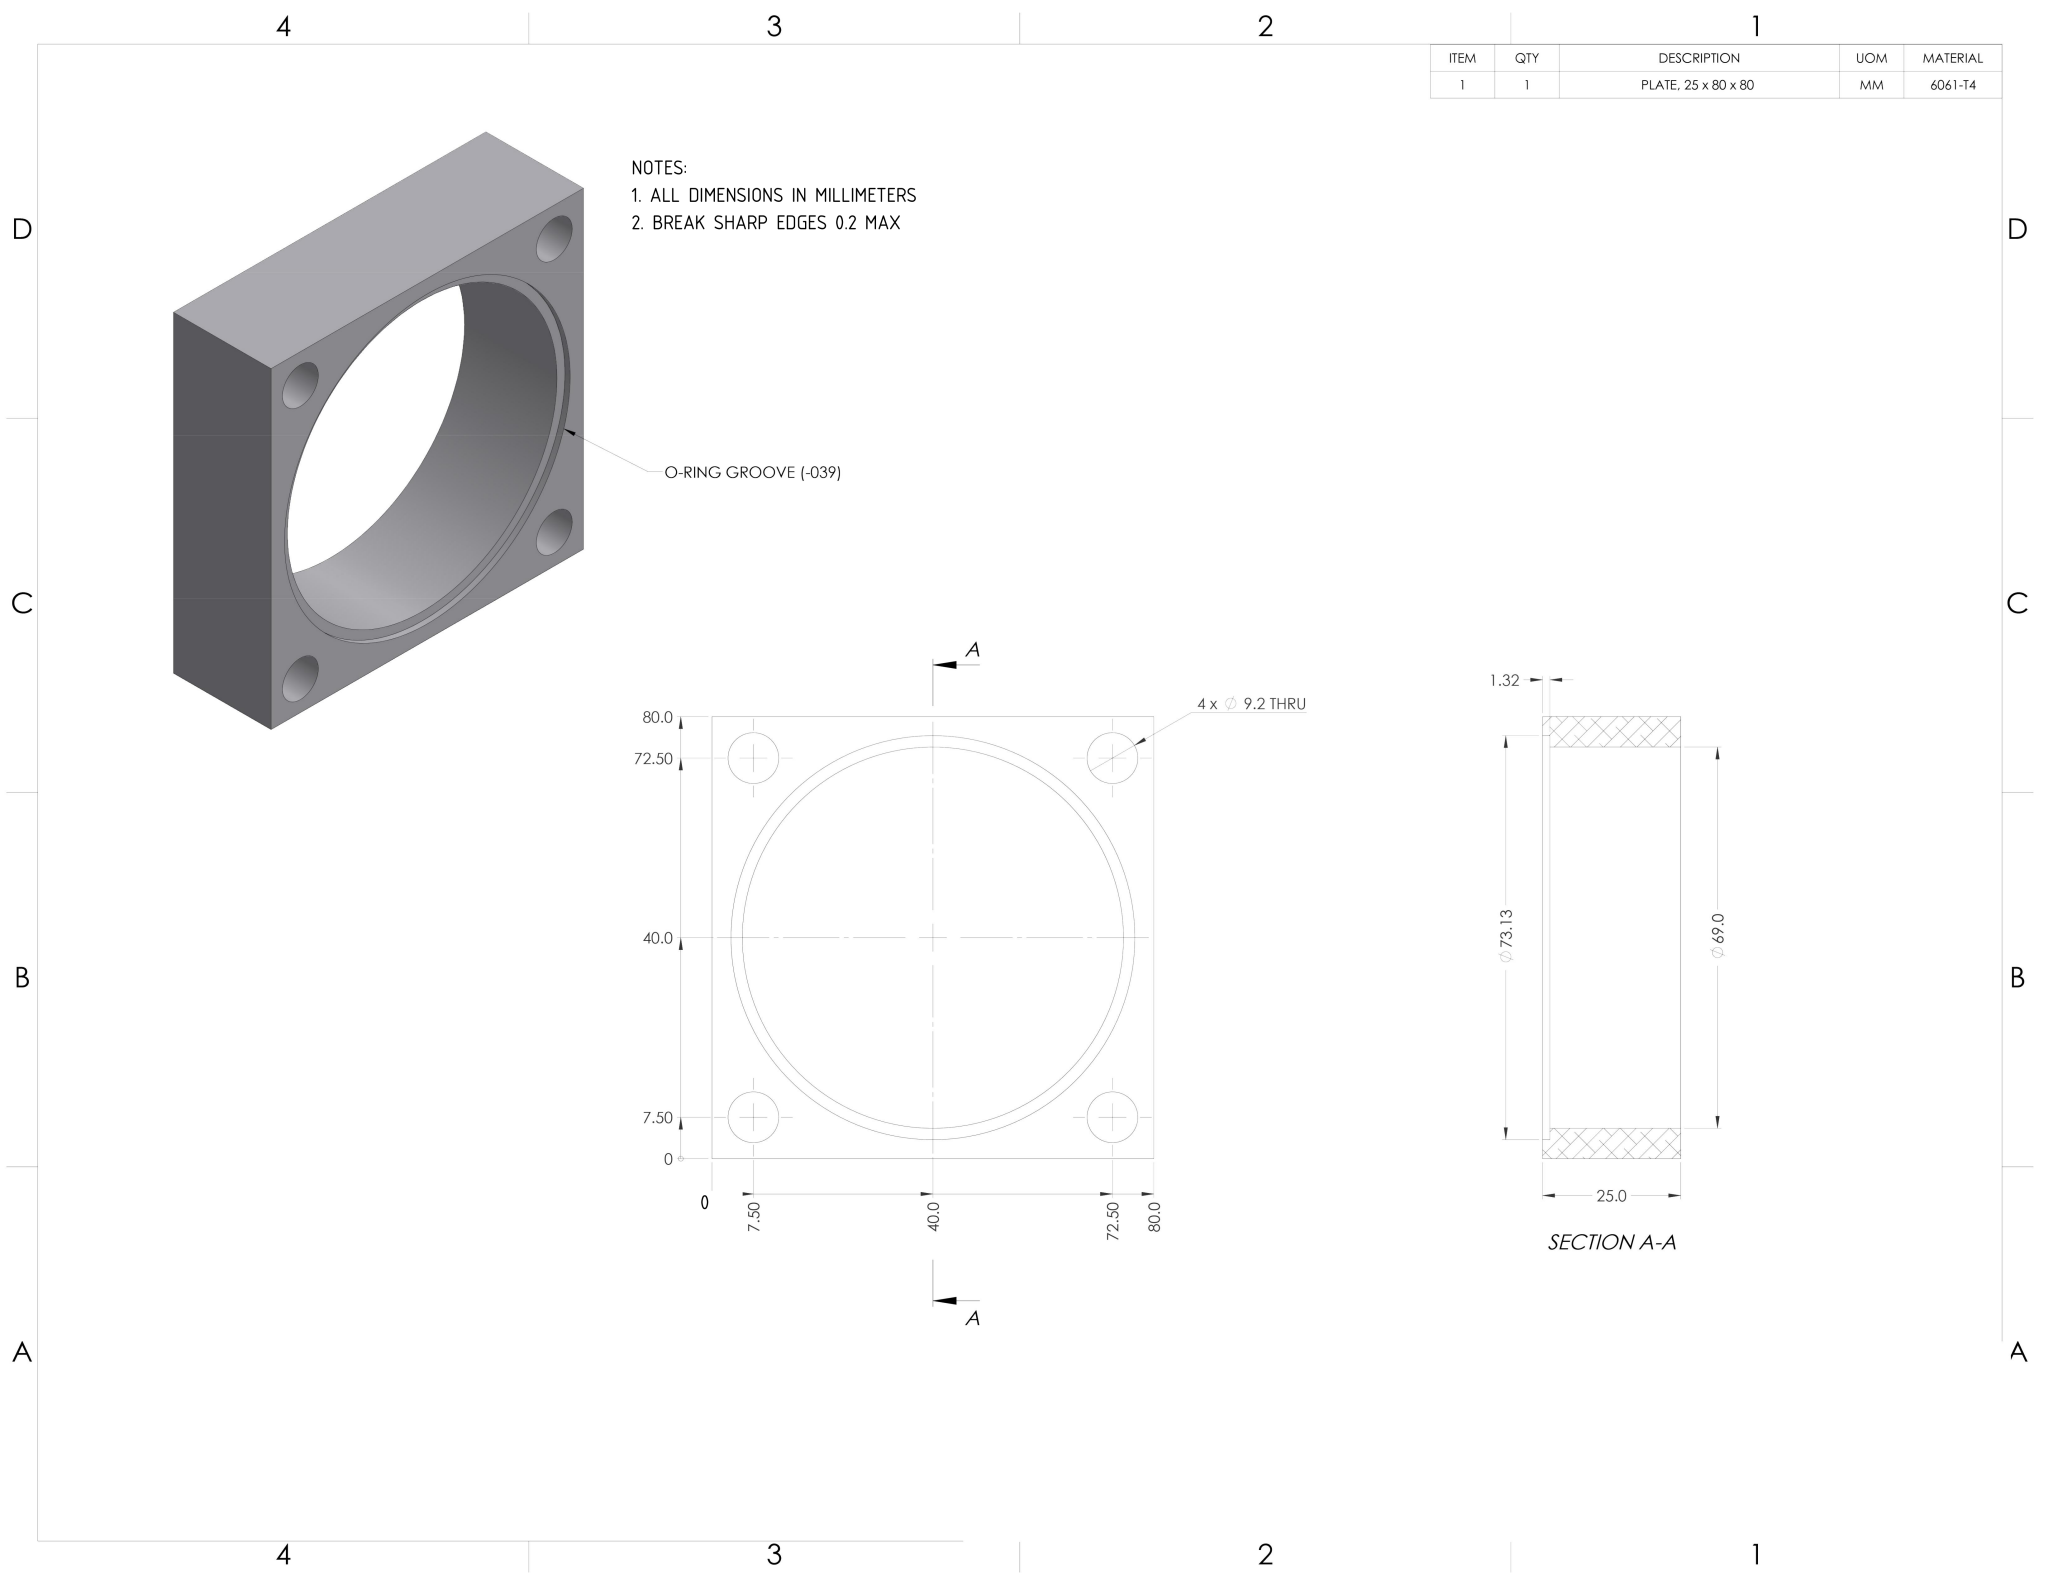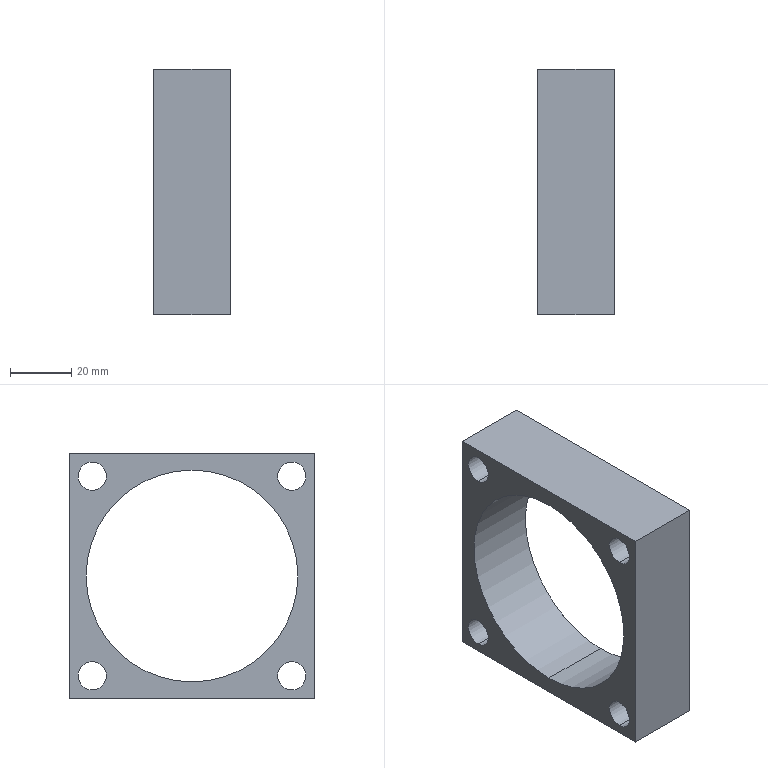Part | NX | mm | Four-Hole Circular Aperture Mounting Bracket | 1 solid | 19 faces | box 25 x 80 x 80 mm | volume 59262 mm3 | cylinder 12 | plane 7 | commonest cylinder face diameters 9.2 x8 69 x2 73.13 x2
STEP:
#1=COLOUR_RGB('',0.8667,0.8667,0.8902);
#2=FILL_AREA_STYLE_COLOUR('',#1);
#3=FILL_AREA_STYLE('',(#2));
#4=SURFACE_STYLE_FILL_AREA(#3);
#5=SURFACE_SIDE_STYLE('',(#4));
#6=SURFACE_STYLE_USAGE(.BOTH.,#5);
#7=PRESENTATION_STYLE_ASSIGNMENT((#6));
#8=CARTESIAN_POINT('',(11.18,0.,34.5));
#9=VERTEX_POINT('',#8);
#10=CARTESIAN_POINT('',(11.18,0.,-34.5));
#11=VERTEX_POINT('',#10);
#12=CARTESIAN_POINT('',(11.18,0.,0.));
#13=DIRECTION('',(1.,0.,0.));
#14=DIRECTION('',(0.,0.,-1.));
#15=AXIS2_PLACEMENT_3D('',#12,#13,#14);
#16=CIRCLE('',#15,34.5);
#17=EDGE_CURVE('',#9,#11,#16,.T.);
#18=ORIENTED_EDGE('',*,*,#17,.T.);
#19=CARTESIAN_POINT('',(-12.5,0.,-34.5));
#20=VERTEX_POINT('',#19);
#21=CARTESIAN_POINT('',(12.501,0.,-34.5));
#22=DIRECTION('',(-1.,0.,0.));
#23=VECTOR('',#22,1000.);
#24=LINE('',#21,#23);
#25=EDGE_CURVE('',#11,#20,#24,.T.);
#26=ORIENTED_EDGE('',*,*,#25,.T.);
#27=CARTESIAN_POINT('',(-12.5,0.,34.5));
#28=VERTEX_POINT('',#27);
#29=CARTESIAN_POINT('',(-12.5,0.,0.));
#30=DIRECTION('',(1.,0.,0.));
#31=DIRECTION('',(0.,0.,-1.));
#32=AXIS2_PLACEMENT_3D('',#29,#30,#31);
#33=CIRCLE('',#32,34.5);
#34=EDGE_CURVE('',#28,#20,#33,.T.);
#35=ORIENTED_EDGE('',*,*,#34,.F.);
#36=CARTESIAN_POINT('',(12.501,0.,34.5));
#37=DIRECTION('',(-1.,0.,0.));
#38=VECTOR('',#37,1000.);
#39=LINE('',#36,#38);
#40=EDGE_CURVE('',#9,#28,#39,.T.);
#41=ORIENTED_EDGE('',*,*,#40,.F.);
#42=EDGE_LOOP('',(#18,#26,#35,#41));
#43=FACE_OUTER_BOUND('',#42,.T.);
#44=CARTESIAN_POINT('',(12.501,0.,0.));
#45=DIRECTION('',(-1.,0.,0.));
#46=DIRECTION('',(0.,0.,1.));
#47=AXIS2_PLACEMENT_3D('',#44,#45,#46);
#48=CYLINDRICAL_SURFACE('',#47,34.5);
#49=ADVANCED_FACE('',(#43),#48,.F.);
#50=CARTESIAN_POINT('',(11.18,0.,36.565));
#51=VERTEX_POINT('',#50);
#52=CARTESIAN_POINT('',(11.18,0.,-36.565));
#53=VERTEX_POINT('',#52);
#54=CARTESIAN_POINT('',(11.18,0.,0.));
#55=DIRECTION('',(1.,0.,0.));
#56=DIRECTION('',(0.,0.,-1.));
#57=AXIS2_PLACEMENT_3D('',#54,#55,#56);
#58=CIRCLE('',#57,36.565);
#59=EDGE_CURVE('',#51,#53,#58,.T.);
#60=ORIENTED_EDGE('',*,*,#59,.F.);
#61=CARTESIAN_POINT('',(12.5,0.,36.565));
#62=VERTEX_POINT('',#61);
#63=CARTESIAN_POINT('',(11.18,0.,36.565));
#64=DIRECTION('',(1.,0.,0.));
#65=VECTOR('',#64,1000.);
#66=LINE('',#63,#65);
#67=EDGE_CURVE('',#51,#62,#66,.T.);
#68=ORIENTED_EDGE('',*,*,#67,.T.);
#69=CARTESIAN_POINT('',(12.5,0.,-36.565));
#70=VERTEX_POINT('',#69);
#71=CARTESIAN_POINT('',(12.5,0.,0.));
#72=DIRECTION('',(1.,0.,0.));
#73=DIRECTION('',(0.,0.,-1.));
#74=AXIS2_PLACEMENT_3D('',#71,#72,#73);
#75=CIRCLE('',#74,36.565);
#76=EDGE_CURVE('',#62,#70,#75,.T.);
#77=ORIENTED_EDGE('',*,*,#76,.T.);
#78=CARTESIAN_POINT('',(11.18,0.,-36.565));
#79=DIRECTION('',(1.,0.,0.));
#80=VECTOR('',#79,1000.);
#81=LINE('',#78,#80);
#82=EDGE_CURVE('',#53,#70,#81,.T.);
#83=ORIENTED_EDGE('',*,*,#82,.F.);
#84=EDGE_LOOP('',(#60,#68,#77,#83));
#85=FACE_OUTER_BOUND('',#84,.T.);
#86=CARTESIAN_POINT('',(11.18,0.,0.));
#87=DIRECTION('',(1.,0.,0.));
#88=DIRECTION('',(0.,0.,-1.));
#89=AXIS2_PLACEMENT_3D('',#86,#87,#88);
#90=CYLINDRICAL_SURFACE('',#89,36.565);
#91=ADVANCED_FACE('',(#85),#90,.F.);
#92=CARTESIAN_POINT('',(12.5,-32.5,37.1));
#93=VERTEX_POINT('',#92);
#94=CARTESIAN_POINT('',(12.5,-32.5,27.9));
#95=VERTEX_POINT('',#94);
#96=CARTESIAN_POINT('',(12.5,-32.5,32.5));
#97=DIRECTION('',(1.,0.,0.));
#98=DIRECTION('',(0.,0.,-1.));
#99=AXIS2_PLACEMENT_3D('',#96,#97,#98);
#100=CIRCLE('',#99,4.6);
#101=EDGE_CURVE('',#93,#95,#100,.T.);
#102=ORIENTED_EDGE('',*,*,#101,.T.);
#103=CARTESIAN_POINT('',(-12.5,-32.5,27.9));
#104=VERTEX_POINT('',#103);
#105=CARTESIAN_POINT('',(-12.5,-32.5,27.9));
#106=DIRECTION('',(-1.,0.,0.));
#107=VECTOR('',#106,1000.);
#108=LINE('',#105,#107);
#109=EDGE_CURVE('',#95,#104,#108,.T.);
#110=ORIENTED_EDGE('',*,*,#109,.T.);
#111=CARTESIAN_POINT('',(-12.5,-32.5,37.1));
#112=VERTEX_POINT('',#111);
#113=CARTESIAN_POINT('',(-12.5,-32.5,32.5));
#114=DIRECTION('',(-1.,0.,0.));
#115=DIRECTION('',(0.,0.,1.));
#116=AXIS2_PLACEMENT_3D('',#113,#114,#115);
#117=CIRCLE('',#116,4.6);
#118=EDGE_CURVE('',#104,#112,#117,.T.);
#119=ORIENTED_EDGE('',*,*,#118,.T.);
#120=CARTESIAN_POINT('',(-12.5,-32.5,37.1));
#121=DIRECTION('',(-1.,0.,0.));
#122=VECTOR('',#121,1000.);
#123=LINE('',#120,#122);
#124=EDGE_CURVE('',#93,#112,#123,.T.);
#125=ORIENTED_EDGE('',*,*,#124,.F.);
#126=EDGE_LOOP('',(#102,#110,#119,#125));
#127=FACE_OUTER_BOUND('',#126,.T.);
#128=CARTESIAN_POINT('',(-12.5,-32.5,32.5));
#129=DIRECTION('',(-1.,0.,0.));
#130=DIRECTION('',(0.,0.,1.));
#131=AXIS2_PLACEMENT_3D('',#128,#129,#130);
#132=CYLINDRICAL_SURFACE('',#131,4.6);
#133=ADVANCED_FACE('',(#127),#132,.F.);
#134=CARTESIAN_POINT('',(12.5,-32.5,-27.9));
#135=VERTEX_POINT('',#134);
#136=CARTESIAN_POINT('',(12.5,-32.5,-37.1));
#137=VERTEX_POINT('',#136);
#138=CARTESIAN_POINT('',(12.5,-32.5,-32.5));
#139=DIRECTION('',(1.,0.,0.));
#140=DIRECTION('',(0.,0.,-1.));
#141=AXIS2_PLACEMENT_3D('',#138,#139,#140);
#142=CIRCLE('',#141,4.6);
#143=EDGE_CURVE('',#135,#137,#142,.T.);
#144=ORIENTED_EDGE('',*,*,#143,.T.);
#145=CARTESIAN_POINT('',(-12.5,-32.5,-37.1));
#146=VERTEX_POINT('',#145);
#147=CARTESIAN_POINT('',(-12.5,-32.5,-37.1));
#148=DIRECTION('',(-1.,0.,0.));
#149=VECTOR('',#148,1000.);
#150=LINE('',#147,#149);
#151=EDGE_CURVE('',#137,#146,#150,.T.);
#152=ORIENTED_EDGE('',*,*,#151,.T.);
#153=CARTESIAN_POINT('',(-12.5,-32.5,-27.9));
#154=VERTEX_POINT('',#153);
#155=CARTESIAN_POINT('',(-12.5,-32.5,-32.5));
#156=DIRECTION('',(-1.,0.,0.));
#157=DIRECTION('',(0.,0.,1.));
#158=AXIS2_PLACEMENT_3D('',#155,#156,#157);
#159=CIRCLE('',#158,4.6);
#160=EDGE_CURVE('',#146,#154,#159,.T.);
#161=ORIENTED_EDGE('',*,*,#160,.T.);
#162=CARTESIAN_POINT('',(-12.5,-32.5,-27.9));
#163=DIRECTION('',(-1.,0.,0.));
#164=VECTOR('',#163,1000.);
#165=LINE('',#162,#164);
#166=EDGE_CURVE('',#135,#154,#165,.T.);
#167=ORIENTED_EDGE('',*,*,#166,.F.);
#168=EDGE_LOOP('',(#144,#152,#161,#167));
#169=FACE_OUTER_BOUND('',#168,.T.);
#170=CARTESIAN_POINT('',(-12.5,-32.5,-32.5));
#171=DIRECTION('',(-1.,0.,0.));
#172=DIRECTION('',(0.,0.,1.));
#173=AXIS2_PLACEMENT_3D('',#170,#171,#172);
#174=CYLINDRICAL_SURFACE('',#173,4.6);
#175=ADVANCED_FACE('',(#169),#174,.F.);
#176=CARTESIAN_POINT('',(12.5,32.5,-27.9));
#177=VERTEX_POINT('',#176);
#178=CARTESIAN_POINT('',(12.5,32.5,-37.1));
#179=VERTEX_POINT('',#178);
#180=CARTESIAN_POINT('',(12.5,32.5,-32.5));
#181=DIRECTION('',(1.,0.,0.));
#182=DIRECTION('',(0.,0.,-1.));
#183=AXIS2_PLACEMENT_3D('',#180,#181,#182);
#184=CIRCLE('',#183,4.6);
#185=EDGE_CURVE('',#177,#179,#184,.T.);
#186=ORIENTED_EDGE('',*,*,#185,.T.);
#187=CARTESIAN_POINT('',(-12.5,32.5,-37.1));
#188=VERTEX_POINT('',#187);
#189=CARTESIAN_POINT('',(-12.5,32.5,-37.1));
#190=DIRECTION('',(-1.,0.,0.));
#191=VECTOR('',#190,1000.);
#192=LINE('',#189,#191);
#193=EDGE_CURVE('',#179,#188,#192,.T.);
#194=ORIENTED_EDGE('',*,*,#193,.T.);
#195=CARTESIAN_POINT('',(-12.5,32.5,-27.9));
#196=VERTEX_POINT('',#195);
#197=CARTESIAN_POINT('',(-12.5,32.5,-32.5));
#198=DIRECTION('',(-1.,0.,0.));
#199=DIRECTION('',(0.,0.,1.));
#200=AXIS2_PLACEMENT_3D('',#197,#198,#199);
#201=CIRCLE('',#200,4.6);
#202=EDGE_CURVE('',#188,#196,#201,.T.);
#203=ORIENTED_EDGE('',*,*,#202,.T.);
#204=CARTESIAN_POINT('',(-12.5,32.5,-27.9));
#205=DIRECTION('',(-1.,0.,0.));
#206=VECTOR('',#205,1000.);
#207=LINE('',#204,#206);
#208=EDGE_CURVE('',#177,#196,#207,.T.);
#209=ORIENTED_EDGE('',*,*,#208,.F.);
#210=EDGE_LOOP('',(#186,#194,#203,#209));
#211=FACE_OUTER_BOUND('',#210,.T.);
#212=CARTESIAN_POINT('',(-12.5,32.5,-32.5));
#213=DIRECTION('',(-1.,0.,0.));
#214=DIRECTION('',(0.,0.,1.));
#215=AXIS2_PLACEMENT_3D('',#212,#213,#214);
#216=CYLINDRICAL_SURFACE('',#215,4.6);
#217=ADVANCED_FACE('',(#211),#216,.F.);
#218=CARTESIAN_POINT('',(12.5,32.5,37.1));
#219=VERTEX_POINT('',#218);
#220=CARTESIAN_POINT('',(12.5,32.5,27.9));
#221=VERTEX_POINT('',#220);
#222=CARTESIAN_POINT('',(12.5,32.5,32.5));
#223=DIRECTION('',(1.,0.,0.));
#224=DIRECTION('',(0.,0.,-1.));
#225=AXIS2_PLACEMENT_3D('',#222,#223,#224);
#226=CIRCLE('',#225,4.6);
#227=EDGE_CURVE('',#219,#221,#226,.T.);
#228=ORIENTED_EDGE('',*,*,#227,.T.);
#229=CARTESIAN_POINT('',(-12.5,32.5,27.9));
#230=VERTEX_POINT('',#229);
#231=CARTESIAN_POINT('',(-12.5,32.5,27.9));
#232=DIRECTION('',(-1.,0.,0.));
#233=VECTOR('',#232,1000.);
#234=LINE('',#231,#233);
#235=EDGE_CURVE('',#221,#230,#234,.T.);
#236=ORIENTED_EDGE('',*,*,#235,.T.);
#237=CARTESIAN_POINT('',(-12.5,32.5,37.1));
#238=VERTEX_POINT('',#237);
#239=CARTESIAN_POINT('',(-12.5,32.5,32.5));
#240=DIRECTION('',(-1.,0.,0.));
#241=DIRECTION('',(0.,0.,1.));
#242=AXIS2_PLACEMENT_3D('',#239,#240,#241);
#243=CIRCLE('',#242,4.6);
#244=EDGE_CURVE('',#230,#238,#243,.T.);
#245=ORIENTED_EDGE('',*,*,#244,.T.);
#246=CARTESIAN_POINT('',(-12.5,32.5,37.1));
#247=DIRECTION('',(-1.,0.,0.));
#248=VECTOR('',#247,1000.);
#249=LINE('',#246,#248);
#250=EDGE_CURVE('',#219,#238,#249,.T.);
#251=ORIENTED_EDGE('',*,*,#250,.F.);
#252=EDGE_LOOP('',(#228,#236,#245,#251));
#253=FACE_OUTER_BOUND('',#252,.T.);
#254=CARTESIAN_POINT('',(-12.5,32.5,32.5));
#255=DIRECTION('',(-1.,0.,0.));
#256=DIRECTION('',(0.,0.,1.));
#257=AXIS2_PLACEMENT_3D('',#254,#255,#256);
#258=CYLINDRICAL_SURFACE('',#257,4.6);
#259=ADVANCED_FACE('',(#253),#258,.F.);
#260=ORIENTED_EDGE('',*,*,#34,.T.);
#261=CARTESIAN_POINT('',(-12.5,0.,0.));
#262=DIRECTION('',(1.,0.,0.));
#263=DIRECTION('',(0.,0.,-1.));
#264=AXIS2_PLACEMENT_3D('',#261,#262,#263);
#265=CIRCLE('',#264,34.5);
#266=EDGE_CURVE('',#20,#28,#265,.T.);
#267=ORIENTED_EDGE('',*,*,#266,.T.);
#268=EDGE_LOOP('',(#260,#267));
#269=FACE_BOUND('',#268,.T.);
#270=CARTESIAN_POINT('',(-12.5,-32.5,-32.5));
#271=DIRECTION('',(-1.,0.,0.));
#272=DIRECTION('',(0.,0.,1.));
#273=AXIS2_PLACEMENT_3D('',#270,#271,#272);
#274=CIRCLE('',#273,4.6);
#275=EDGE_CURVE('',#154,#146,#274,.T.);
#276=ORIENTED_EDGE('',*,*,#275,.F.);
#277=ORIENTED_EDGE('',*,*,#160,.F.);
#278=EDGE_LOOP('',(#276,#277));
#279=FACE_BOUND('',#278,.T.);
#280=CARTESIAN_POINT('',(-12.5,32.5,-32.5));
#281=DIRECTION('',(-1.,0.,0.));
#282=DIRECTION('',(0.,0.,1.));
#283=AXIS2_PLACEMENT_3D('',#280,#281,#282);
#284=CIRCLE('',#283,4.6);
#285=EDGE_CURVE('',#196,#188,#284,.T.);
#286=ORIENTED_EDGE('',*,*,#285,.F.);
#287=ORIENTED_EDGE('',*,*,#202,.F.);
#288=EDGE_LOOP('',(#286,#287));
#289=FACE_BOUND('',#288,.T.);
#290=CARTESIAN_POINT('',(-12.5,32.5,32.5));
#291=DIRECTION('',(-1.,0.,0.));
#292=DIRECTION('',(0.,0.,1.));
#293=AXIS2_PLACEMENT_3D('',#290,#291,#292);
#294=CIRCLE('',#293,4.6);
#295=EDGE_CURVE('',#238,#230,#294,.T.);
#296=ORIENTED_EDGE('',*,*,#295,.F.);
#297=ORIENTED_EDGE('',*,*,#244,.F.);
#298=EDGE_LOOP('',(#296,#297));
#299=FACE_BOUND('',#298,.T.);
#300=CARTESIAN_POINT('',(-12.5,40.,40.));
#301=VERTEX_POINT('',#300);
#302=CARTESIAN_POINT('',(-12.5,-40.,40.));
#303=VERTEX_POINT('',#302);
#304=CARTESIAN_POINT('',(-12.5,40.,40.));
#305=DIRECTION('',(0.,-1.,-0.));
#306=VECTOR('',#305,1000.);
#307=LINE('',#304,#306);
#308=EDGE_CURVE('',#301,#303,#307,.T.);
#309=ORIENTED_EDGE('',*,*,#308,.F.);
#310=CARTESIAN_POINT('',(-12.5,40.,-40.));
#311=VERTEX_POINT('',#310);
#312=CARTESIAN_POINT('',(-12.5,40.,40.));
#313=DIRECTION('',(0.,0.,1.));
#314=VECTOR('',#313,1000.);
#315=LINE('',#312,#314);
#316=EDGE_CURVE('',#311,#301,#315,.T.);
#317=ORIENTED_EDGE('',*,*,#316,.F.);
#318=CARTESIAN_POINT('',(-12.5,-40.,-40.));
#319=VERTEX_POINT('',#318);
#320=CARTESIAN_POINT('',(-12.5,40.,-40.));
#321=DIRECTION('',(0.,1.,-0.));
#322=VECTOR('',#321,1000.);
#323=LINE('',#320,#322);
#324=EDGE_CURVE('',#319,#311,#323,.T.);
#325=ORIENTED_EDGE('',*,*,#324,.F.);
#326=CARTESIAN_POINT('',(-12.5,-40.,40.));
#327=DIRECTION('',(0.,0.,-1.));
#328=VECTOR('',#327,1000.);
#329=LINE('',#326,#328);
#330=EDGE_CURVE('',#303,#319,#329,.T.);
#331=ORIENTED_EDGE('',*,*,#330,.F.);
#332=EDGE_LOOP('',(#309,#317,#325,#331));
#333=FACE_OUTER_BOUND('',#332,.T.);
#334=CARTESIAN_POINT('',(-12.5,-32.5,32.5));
#335=DIRECTION('',(-1.,0.,0.));
#336=DIRECTION('',(0.,0.,1.));
#337=AXIS2_PLACEMENT_3D('',#334,#335,#336);
#338=CIRCLE('',#337,4.6);
#339=EDGE_CURVE('',#112,#104,#338,.T.);
#340=ORIENTED_EDGE('',*,*,#339,.F.);
#341=ORIENTED_EDGE('',*,*,#118,.F.);
#342=EDGE_LOOP('',(#340,#341));
#343=FACE_BOUND('',#342,.T.);
#344=CARTESIAN_POINT('',(-12.5,0.,0.));
#345=DIRECTION('',(1.,0.,0.));
#346=DIRECTION('',(0.,0.,-1.));
#347=AXIS2_PLACEMENT_3D('',#344,#345,#346);
#348=PLANE('',#347);
#349=ADVANCED_FACE('',(#269,#279,#289,#299,#333,#343),#348,.F.);
#350=ORIENTED_EDGE('',*,*,#308,.T.);
#351=CARTESIAN_POINT('',(12.5,-40.,40.));
#352=VERTEX_POINT('',#351);
#353=CARTESIAN_POINT('',(12.5,-40.,40.));
#354=DIRECTION('',(-1.,0.,0.));
#355=VECTOR('',#354,1000.);
#356=LINE('',#353,#355);
#357=EDGE_CURVE('',#352,#303,#356,.T.);
#358=ORIENTED_EDGE('',*,*,#357,.F.);
#359=CARTESIAN_POINT('',(12.5,40.,40.));
#360=VERTEX_POINT('',#359);
#361=CARTESIAN_POINT('',(12.5,40.,40.));
#362=DIRECTION('',(0.,-1.,-0.));
#363=VECTOR('',#362,1000.);
#364=LINE('',#361,#363);
#365=EDGE_CURVE('',#360,#352,#364,.T.);
#366=ORIENTED_EDGE('',*,*,#365,.F.);
#367=CARTESIAN_POINT('',(12.5,40.,40.));
#368=DIRECTION('',(-1.,0.,0.));
#369=VECTOR('',#368,1000.);
#370=LINE('',#367,#369);
#371=EDGE_CURVE('',#360,#301,#370,.T.);
#372=ORIENTED_EDGE('',*,*,#371,.T.);
#373=EDGE_LOOP('',(#350,#358,#366,#372));
#374=FACE_OUTER_BOUND('',#373,.T.);
#375=CARTESIAN_POINT('',(12.5,40.,40.));
#376=DIRECTION('',(0.,0.,-1.));
#377=DIRECTION('',(0.,1.,0.));
#378=AXIS2_PLACEMENT_3D('',#375,#376,#377);
#379=PLANE('',#378);
#380=ADVANCED_FACE('',(#374),#379,.F.);
#381=ORIENTED_EDGE('',*,*,#330,.T.);
#382=CARTESIAN_POINT('',(12.5,-40.,-40.));
#383=VERTEX_POINT('',#382);
#384=CARTESIAN_POINT('',(12.5,-40.,-40.));
#385=DIRECTION('',(-1.,0.,0.));
#386=VECTOR('',#385,1000.);
#387=LINE('',#384,#386);
#388=EDGE_CURVE('',#383,#319,#387,.T.);
#389=ORIENTED_EDGE('',*,*,#388,.F.);
#390=CARTESIAN_POINT('',(12.5,-40.,40.));
#391=DIRECTION('',(0.,0.,-1.));
#392=VECTOR('',#391,1000.);
#393=LINE('',#390,#392);
#394=EDGE_CURVE('',#352,#383,#393,.T.);
#395=ORIENTED_EDGE('',*,*,#394,.F.);
#396=ORIENTED_EDGE('',*,*,#357,.T.);
#397=EDGE_LOOP('',(#381,#389,#395,#396));
#398=FACE_OUTER_BOUND('',#397,.T.);
#399=CARTESIAN_POINT('',(12.5,-40.,40.));
#400=DIRECTION('',(0.,1.,0.));
#401=DIRECTION('',(0.,0.,1.));
#402=AXIS2_PLACEMENT_3D('',#399,#400,#401);
#403=PLANE('',#402);
#404=ADVANCED_FACE('',(#398),#403,.F.);
#405=ORIENTED_EDGE('',*,*,#324,.T.);
#406=CARTESIAN_POINT('',(12.5,40.,-40.));
#407=VERTEX_POINT('',#406);
#408=CARTESIAN_POINT('',(12.5,40.,-40.));
#409=DIRECTION('',(-1.,0.,0.));
#410=VECTOR('',#409,1000.);
#411=LINE('',#408,#410);
#412=EDGE_CURVE('',#407,#311,#411,.T.);
#413=ORIENTED_EDGE('',*,*,#412,.F.);
#414=CARTESIAN_POINT('',(12.5,40.,-40.));
#415=DIRECTION('',(0.,1.,-0.));
#416=VECTOR('',#415,1000.);
#417=LINE('',#414,#416);
#418=EDGE_CURVE('',#383,#407,#417,.T.);
#419=ORIENTED_EDGE('',*,*,#418,.F.);
#420=ORIENTED_EDGE('',*,*,#388,.T.);
#421=EDGE_LOOP('',(#405,#413,#419,#420));
#422=FACE_OUTER_BOUND('',#421,.T.);
#423=CARTESIAN_POINT('',(12.5,40.,-40.));
#424=DIRECTION('',(0.,0.,1.));
#425=DIRECTION('',(0.,-1.,0.));
#426=AXIS2_PLACEMENT_3D('',#423,#424,#425);
#427=PLANE('',#426);
#428=ADVANCED_FACE('',(#422),#427,.F.);
#429=ORIENTED_EDGE('',*,*,#316,.T.);
#430=ORIENTED_EDGE('',*,*,#371,.F.);
#431=CARTESIAN_POINT('',(12.5,40.,40.));
#432=DIRECTION('',(0.,0.,1.));
#433=VECTOR('',#432,1000.);
#434=LINE('',#431,#433);
#435=EDGE_CURVE('',#407,#360,#434,.T.);
#436=ORIENTED_EDGE('',*,*,#435,.F.);
#437=ORIENTED_EDGE('',*,*,#412,.T.);
#438=EDGE_LOOP('',(#429,#430,#436,#437));
#439=FACE_OUTER_BOUND('',#438,.T.);
#440=CARTESIAN_POINT('',(12.5,40.,40.));
#441=DIRECTION('',(0.,-1.,0.));
#442=DIRECTION('',(0.,0.,-1.));
#443=AXIS2_PLACEMENT_3D('',#440,#441,#442);
#444=PLANE('',#443);
#445=ADVANCED_FACE('',(#439),#444,.F.);
#446=CARTESIAN_POINT('',(12.5,0.,0.));
#447=DIRECTION('',(1.,0.,0.));
#448=DIRECTION('',(0.,0.,-1.));
#449=AXIS2_PLACEMENT_3D('',#446,#447,#448);
#450=CIRCLE('',#449,36.565);
#451=EDGE_CURVE('',#70,#62,#450,.T.);
#452=ORIENTED_EDGE('',*,*,#451,.F.);
#453=ORIENTED_EDGE('',*,*,#76,.F.);
#454=EDGE_LOOP('',(#452,#453));
#455=FACE_BOUND('',#454,.T.);
#456=ORIENTED_EDGE('',*,*,#101,.F.);
#457=CARTESIAN_POINT('',(12.5,-32.5,32.5));
#458=DIRECTION('',(1.,0.,0.));
#459=DIRECTION('',(0.,0.,-1.));
#460=AXIS2_PLACEMENT_3D('',#457,#458,#459);
#461=CIRCLE('',#460,4.6);
#462=EDGE_CURVE('',#95,#93,#461,.T.);
#463=ORIENTED_EDGE('',*,*,#462,.F.);
#464=EDGE_LOOP('',(#456,#463));
#465=FACE_BOUND('',#464,.T.);
#466=ORIENTED_EDGE('',*,*,#143,.F.);
#467=CARTESIAN_POINT('',(12.5,-32.5,-32.5));
#468=DIRECTION('',(1.,0.,0.));
#469=DIRECTION('',(0.,0.,-1.));
#470=AXIS2_PLACEMENT_3D('',#467,#468,#469);
#471=CIRCLE('',#470,4.6);
#472=EDGE_CURVE('',#137,#135,#471,.T.);
#473=ORIENTED_EDGE('',*,*,#472,.F.);
#474=EDGE_LOOP('',(#466,#473));
#475=FACE_BOUND('',#474,.T.);
#476=ORIENTED_EDGE('',*,*,#185,.F.);
#477=CARTESIAN_POINT('',(12.5,32.5,-32.5));
#478=DIRECTION('',(1.,0.,0.));
#479=DIRECTION('',(0.,0.,-1.));
#480=AXIS2_PLACEMENT_3D('',#477,#478,#479);
#481=CIRCLE('',#480,4.6);
#482=EDGE_CURVE('',#179,#177,#481,.T.);
#483=ORIENTED_EDGE('',*,*,#482,.F.);
#484=EDGE_LOOP('',(#476,#483));
#485=FACE_BOUND('',#484,.T.);
#486=ORIENTED_EDGE('',*,*,#227,.F.);
#487=CARTESIAN_POINT('',(12.5,32.5,32.5));
#488=DIRECTION('',(1.,0.,0.));
#489=DIRECTION('',(0.,0.,-1.));
#490=AXIS2_PLACEMENT_3D('',#487,#488,#489);
#491=CIRCLE('',#490,4.6);
#492=EDGE_CURVE('',#221,#219,#491,.T.);
#493=ORIENTED_EDGE('',*,*,#492,.F.);
#494=EDGE_LOOP('',(#486,#493));
#495=FACE_BOUND('',#494,.T.);
#496=ORIENTED_EDGE('',*,*,#365,.T.);
#497=ORIENTED_EDGE('',*,*,#394,.T.);
#498=ORIENTED_EDGE('',*,*,#418,.T.);
#499=ORIENTED_EDGE('',*,*,#435,.T.);
#500=EDGE_LOOP('',(#496,#497,#498,#499));
#501=FACE_OUTER_BOUND('',#500,.T.);
#502=CARTESIAN_POINT('',(12.5,0.,0.));
#503=DIRECTION('',(1.,0.,0.));
#504=DIRECTION('',(0.,0.,-1.));
#505=AXIS2_PLACEMENT_3D('',#502,#503,#504);
#506=PLANE('',#505);
#507=ADVANCED_FACE('',(#455,#465,#475,#485,#495,#501),#506,.T.);
#508=ORIENTED_EDGE('',*,*,#235,.F.);
#509=ORIENTED_EDGE('',*,*,#492,.T.);
#510=ORIENTED_EDGE('',*,*,#250,.T.);
#511=ORIENTED_EDGE('',*,*,#295,.T.);
#512=EDGE_LOOP('',(#508,#509,#510,#511));
#513=FACE_OUTER_BOUND('',#512,.T.);
#514=CARTESIAN_POINT('',(-12.5,32.5,32.5));
#515=DIRECTION('',(-1.,0.,0.));
#516=DIRECTION('',(0.,0.,1.));
#517=AXIS2_PLACEMENT_3D('',#514,#515,#516);
#518=CYLINDRICAL_SURFACE('',#517,4.6);
#519=ADVANCED_FACE('',(#513),#518,.F.);
#520=ORIENTED_EDGE('',*,*,#193,.F.);
#521=ORIENTED_EDGE('',*,*,#482,.T.);
#522=ORIENTED_EDGE('',*,*,#208,.T.);
#523=ORIENTED_EDGE('',*,*,#285,.T.);
#524=EDGE_LOOP('',(#520,#521,#522,#523));
#525=FACE_OUTER_BOUND('',#524,.T.);
#526=CARTESIAN_POINT('',(-12.5,32.5,-32.5));
#527=DIRECTION('',(-1.,0.,0.));
#528=DIRECTION('',(0.,0.,1.));
#529=AXIS2_PLACEMENT_3D('',#526,#527,#528);
#530=CYLINDRICAL_SURFACE('',#529,4.6);
#531=ADVANCED_FACE('',(#525),#530,.F.);
#532=ORIENTED_EDGE('',*,*,#151,.F.);
#533=ORIENTED_EDGE('',*,*,#472,.T.);
#534=ORIENTED_EDGE('',*,*,#166,.T.);
#535=ORIENTED_EDGE('',*,*,#275,.T.);
#536=EDGE_LOOP('',(#532,#533,#534,#535));
#537=FACE_OUTER_BOUND('',#536,.T.);
#538=CARTESIAN_POINT('',(-12.5,-32.5,-32.5));
#539=DIRECTION('',(-1.,0.,0.));
#540=DIRECTION('',(0.,0.,1.));
#541=AXIS2_PLACEMENT_3D('',#538,#539,#540);
#542=CYLINDRICAL_SURFACE('',#541,4.6);
#543=ADVANCED_FACE('',(#537),#542,.F.);
#544=ORIENTED_EDGE('',*,*,#109,.F.);
#545=ORIENTED_EDGE('',*,*,#462,.T.);
#546=ORIENTED_EDGE('',*,*,#124,.T.);
#547=ORIENTED_EDGE('',*,*,#339,.T.);
#548=EDGE_LOOP('',(#544,#545,#546,#547));
#549=FACE_OUTER_BOUND('',#548,.T.);
#550=CARTESIAN_POINT('',(-12.5,-32.5,32.5));
#551=DIRECTION('',(-1.,0.,0.));
#552=DIRECTION('',(0.,0.,1.));
#553=AXIS2_PLACEMENT_3D('',#550,#551,#552);
#554=CYLINDRICAL_SURFACE('',#553,4.6);
#555=ADVANCED_FACE('',(#549),#554,.F.);
#556=ORIENTED_EDGE('',*,*,#67,.F.);
#557=CARTESIAN_POINT('',(11.18,0.,0.));
#558=DIRECTION('',(1.,0.,0.));
#559=DIRECTION('',(0.,0.,-1.));
#560=AXIS2_PLACEMENT_3D('',#557,#558,#559);
#561=CIRCLE('',#560,36.565);
#562=EDGE_CURVE('',#53,#51,#561,.T.);
#563=ORIENTED_EDGE('',*,*,#562,.F.);
#564=ORIENTED_EDGE('',*,*,#82,.T.);
#565=ORIENTED_EDGE('',*,*,#451,.T.);
#566=EDGE_LOOP('',(#556,#563,#564,#565));
#567=FACE_OUTER_BOUND('',#566,.T.);
#568=CARTESIAN_POINT('',(11.18,0.,0.));
#569=DIRECTION('',(1.,0.,0.));
#570=DIRECTION('',(0.,0.,-1.));
#571=AXIS2_PLACEMENT_3D('',#568,#569,#570);
#572=CYLINDRICAL_SURFACE('',#571,36.565);
#573=ADVANCED_FACE('',(#567),#572,.F.);
#574=ORIENTED_EDGE('',*,*,#17,.F.);
#575=CARTESIAN_POINT('',(11.18,0.,0.));
#576=DIRECTION('',(1.,0.,0.));
#577=DIRECTION('',(0.,0.,-1.));
#578=AXIS2_PLACEMENT_3D('',#575,#576,#577);
#579=CIRCLE('',#578,34.5);
#580=EDGE_CURVE('',#11,#9,#579,.T.);
#581=ORIENTED_EDGE('',*,*,#580,.F.);
#582=EDGE_LOOP('',(#574,#581));
#583=FACE_BOUND('',#582,.T.);
#584=ORIENTED_EDGE('',*,*,#562,.T.);
#585=ORIENTED_EDGE('',*,*,#59,.T.);
#586=EDGE_LOOP('',(#584,#585));
#587=FACE_OUTER_BOUND('',#586,.T.);
#588=CARTESIAN_POINT('',(11.18,0.,0.));
#589=DIRECTION('',(1.,0.,0.));
#590=DIRECTION('',(0.,0.,-1.));
#591=AXIS2_PLACEMENT_3D('',#588,#589,#590);
#592=PLANE('',#591);
#593=ADVANCED_FACE('',(#583,#587),#592,.T.);
#594=ORIENTED_EDGE('',*,*,#25,.F.);
#595=ORIENTED_EDGE('',*,*,#580,.T.);
#596=ORIENTED_EDGE('',*,*,#40,.T.);
#597=ORIENTED_EDGE('',*,*,#266,.F.);
#598=EDGE_LOOP('',(#594,#595,#596,#597));
#599=FACE_OUTER_BOUND('',#598,.T.);
#600=CARTESIAN_POINT('',(12.501,0.,0.));
#601=DIRECTION('',(-1.,0.,0.));
#602=DIRECTION('',(0.,0.,1.));
#603=AXIS2_PLACEMENT_3D('',#600,#601,#602);
#604=CYLINDRICAL_SURFACE('',#603,34.5);
#605=ADVANCED_FACE('',(#599),#604,.F.);
#606=CLOSED_SHELL('',(#49,#91,#133,#175,#217,#259,#349,#380,#404,#428,#445,#507,#519,#531,#543,#555,#573,#593,#605));
#607=MANIFOLD_SOLID_BREP('',#606);
#608=STYLED_ITEM('',(#7),#607);
#609=PRESENTATION_LAYER_ASSIGNMENT('','',(#608));
#610=COLOUR_RGB('',0.8667,0.8667,0.8902);
#611=FILL_AREA_STYLE_COLOUR('',#610);
#612=FILL_AREA_STYLE('',(#611));
#613=SURFACE_STYLE_FILL_AREA(#612);
#614=SURFACE_SIDE_STYLE('',(#613));
#615=SURFACE_STYLE_USAGE(.BOTH.,#614);
#616=PRESENTATION_STYLE_ASSIGNMENT((#615));
#617=CARTESIAN_POINT('',(0.,0.,0.));
#618=DIRECTION('',(0.,0.,1.));
#619=DIRECTION('',(1.,0.,0.));
#620=AXIS2_PLACEMENT_3D('',#617,#618,#619);
#621=(LENGTH_UNIT()NAMED_UNIT(*)SI_UNIT(.MILLI.,.METRE.));
#622=UNCERTAINTY_MEASURE_WITH_UNIT(LENGTH_MEASURE(0.00001),#621,'','');
#623=(NAMED_UNIT(*)PLANE_ANGLE_UNIT()SI_UNIT($,.RADIAN.));
#624=(NAMED_UNIT(*)SI_UNIT($,.STERADIAN.)SOLID_ANGLE_UNIT());
#625=(GEOMETRIC_REPRESENTATION_CONTEXT(3)GLOBAL_UNCERTAINTY_ASSIGNED_CONTEXT((#622))GLOBAL_UNIT_ASSIGNED_CONTEXT((#621,#623,#624))REPRESENTATION_CONTEXT('',''));
#626=ADVANCED_BREP_SHAPE_REPRESENTATION('',(#607,#620),#625);
#627=STYLED_ITEM('',(#616),#626);
#628=(LENGTH_UNIT()NAMED_UNIT(*)SI_UNIT(.MILLI.,.METRE.));
#629=UNCERTAINTY_MEASURE_WITH_UNIT(LENGTH_MEASURE(0.00001),#628,'','');
#630=(NAMED_UNIT(*)PLANE_ANGLE_UNIT()SI_UNIT($,.RADIAN.));
#631=(NAMED_UNIT(*)SI_UNIT($,.STERADIAN.)SOLID_ANGLE_UNIT());
#632=(GEOMETRIC_REPRESENTATION_CONTEXT(3)GLOBAL_UNCERTAINTY_ASSIGNED_CONTEXT((#629))GLOBAL_UNIT_ASSIGNED_CONTEXT((#628,#630,#631))REPRESENTATION_CONTEXT('',''));
#633=MECHANICAL_DESIGN_GEOMETRIC_PRESENTATION_REPRESENTATION('',(#627),#632);
#634=(LENGTH_UNIT()NAMED_UNIT(*)SI_UNIT(.MILLI.,.METRE.));
#635=UNCERTAINTY_MEASURE_WITH_UNIT(LENGTH_MEASURE(0.00001),#634,'','');
#636=(NAMED_UNIT(*)PLANE_ANGLE_UNIT()SI_UNIT($,.RADIAN.));
#637=(NAMED_UNIT(*)SI_UNIT($,.STERADIAN.)SOLID_ANGLE_UNIT());
#638=(GEOMETRIC_REPRESENTATION_CONTEXT(3)GLOBAL_UNCERTAINTY_ASSIGNED_CONTEXT((#635))GLOBAL_UNIT_ASSIGNED_CONTEXT((#634,#636,#637))REPRESENTATION_CONTEXT('',''));
#639=MECHANICAL_DESIGN_GEOMETRIC_PRESENTATION_REPRESENTATION('',(#608),#638);
#640=PRESENTATION_LAYER_ASSIGNMENT('','',(#627));